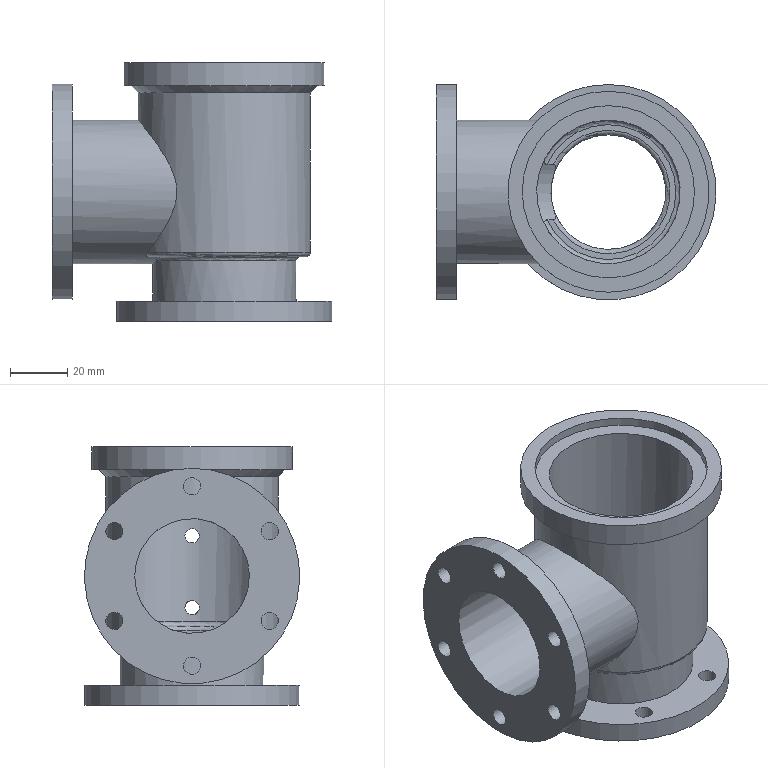Component | NX | VALVE_BODY | 1 solid | 38 faces | volume 133613 mm3 | cylinder 24 | plane 9 | torus 4 | cone 1 | commonest cylinder face diameters 6 x12 50 x3 60 x2 40 x2 75 x2 5 x2 70 x1